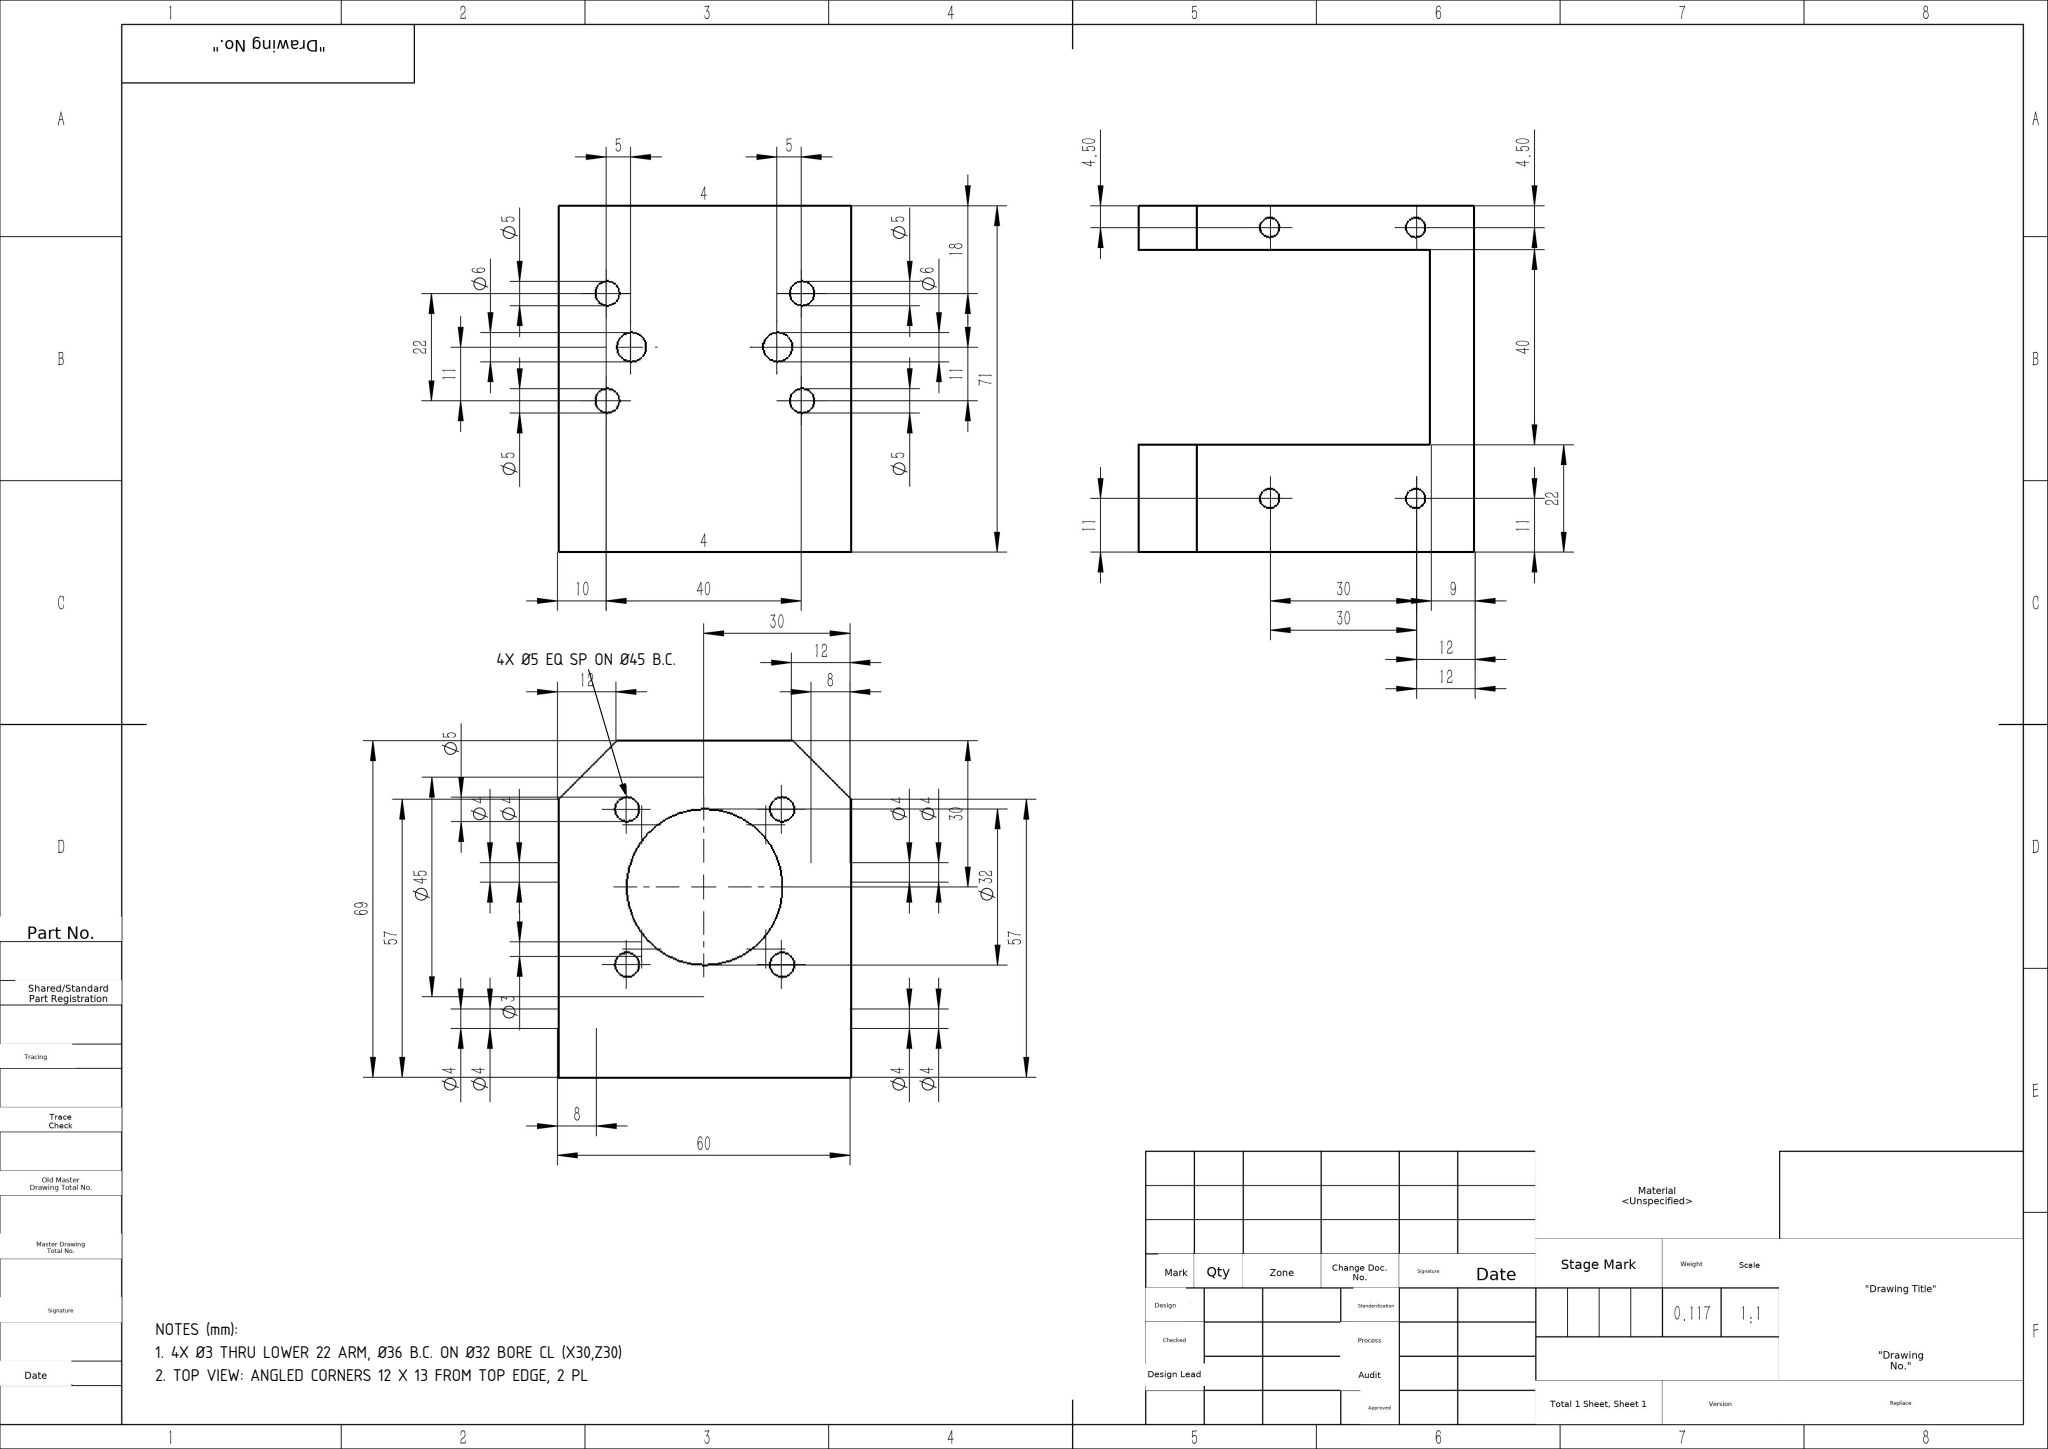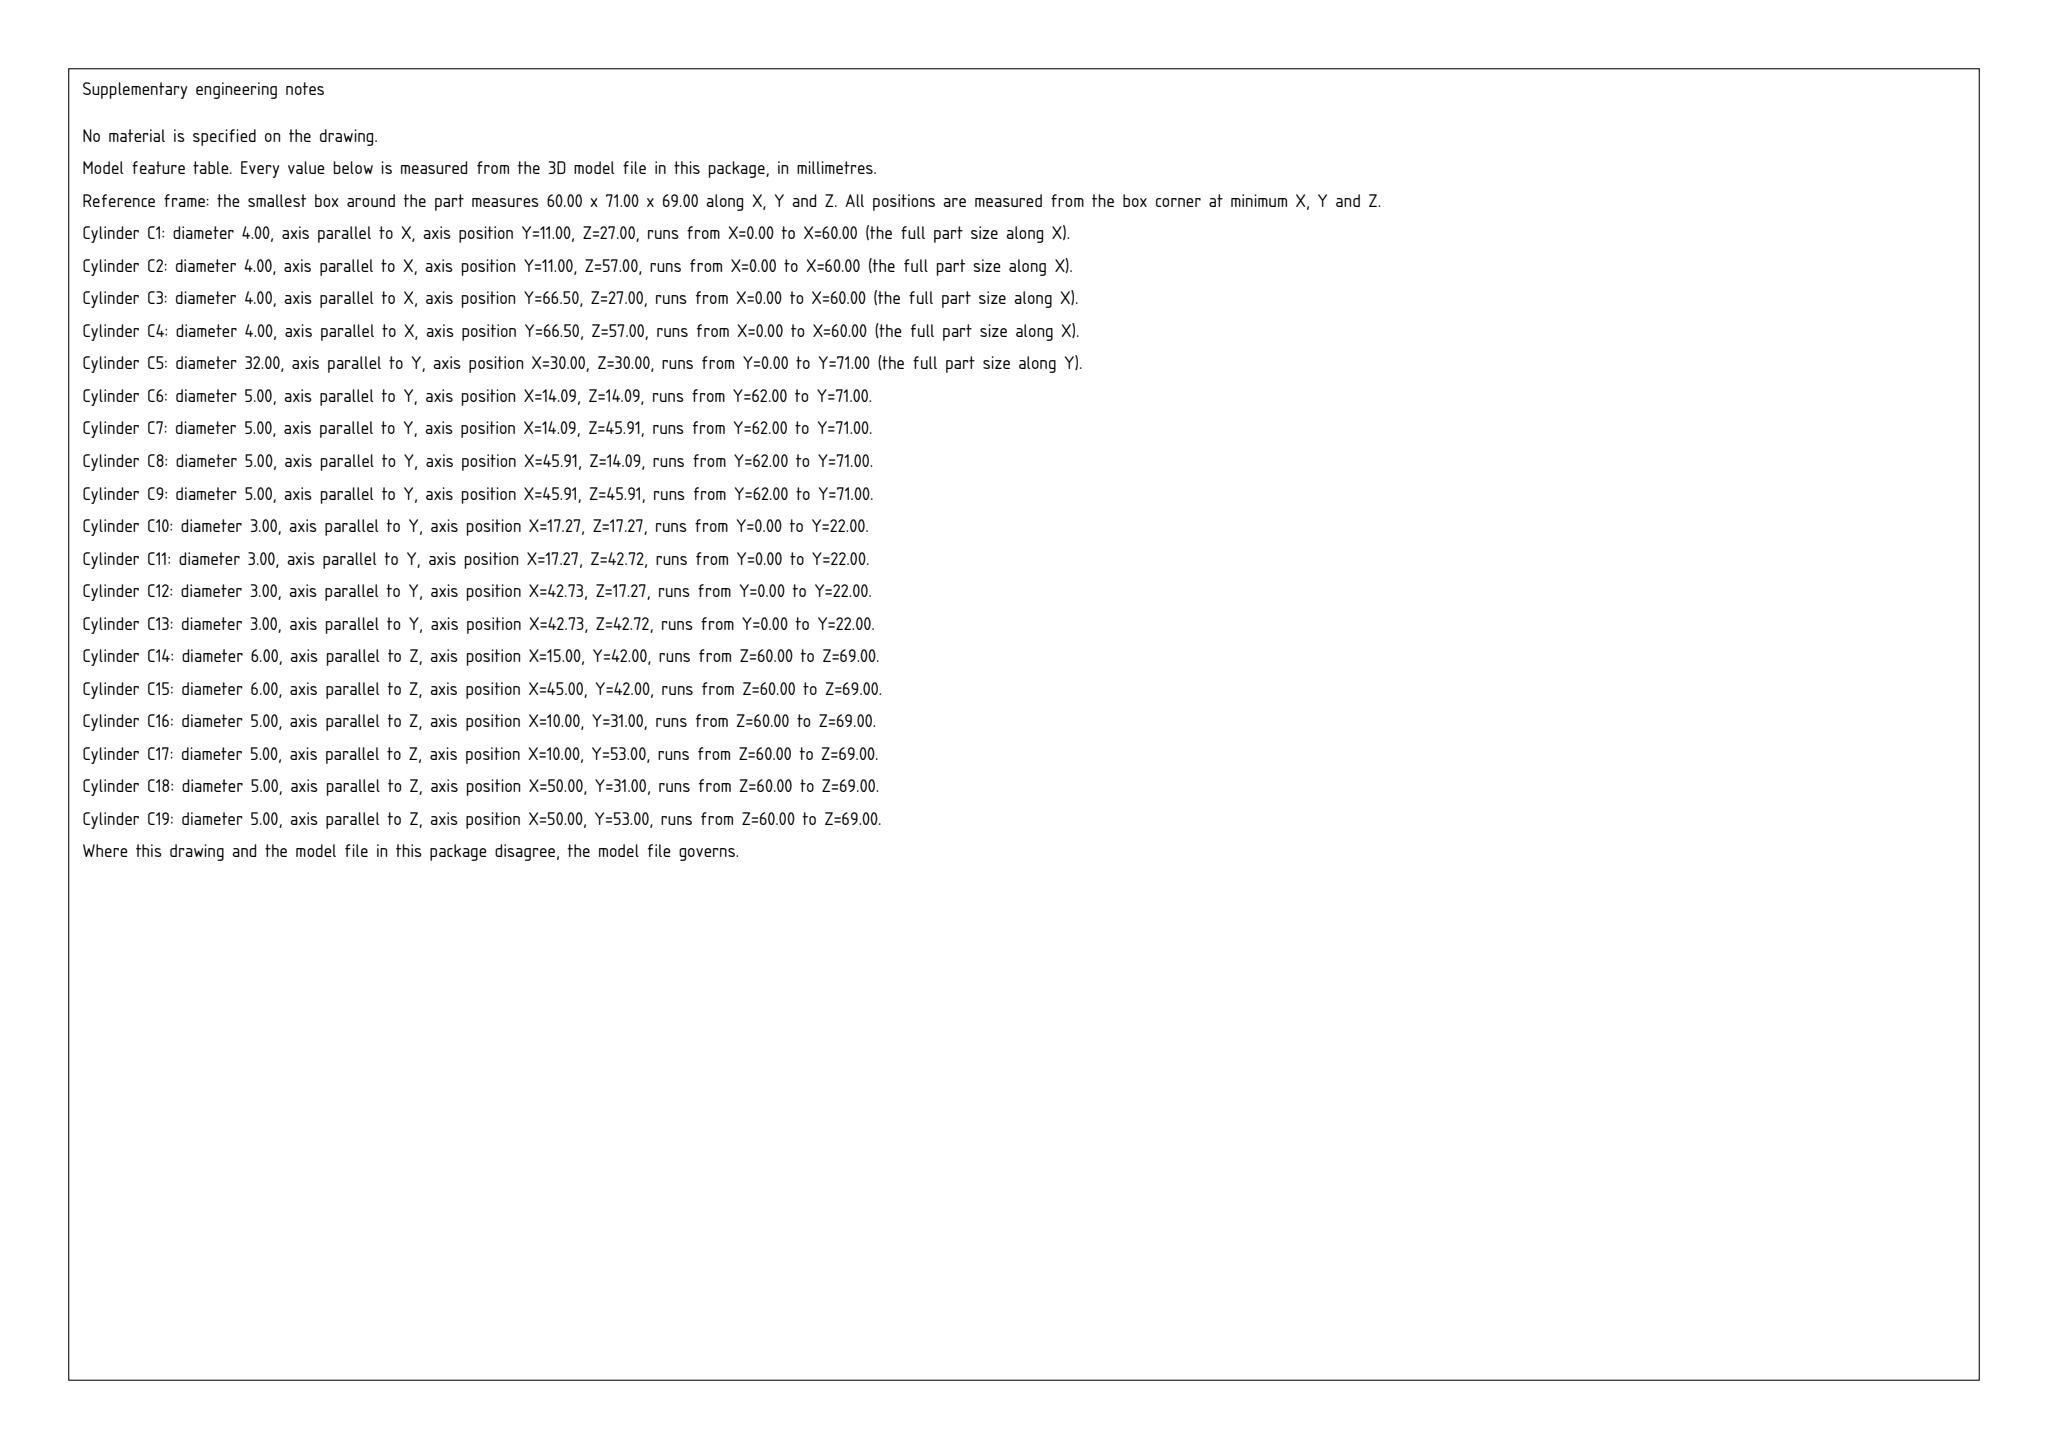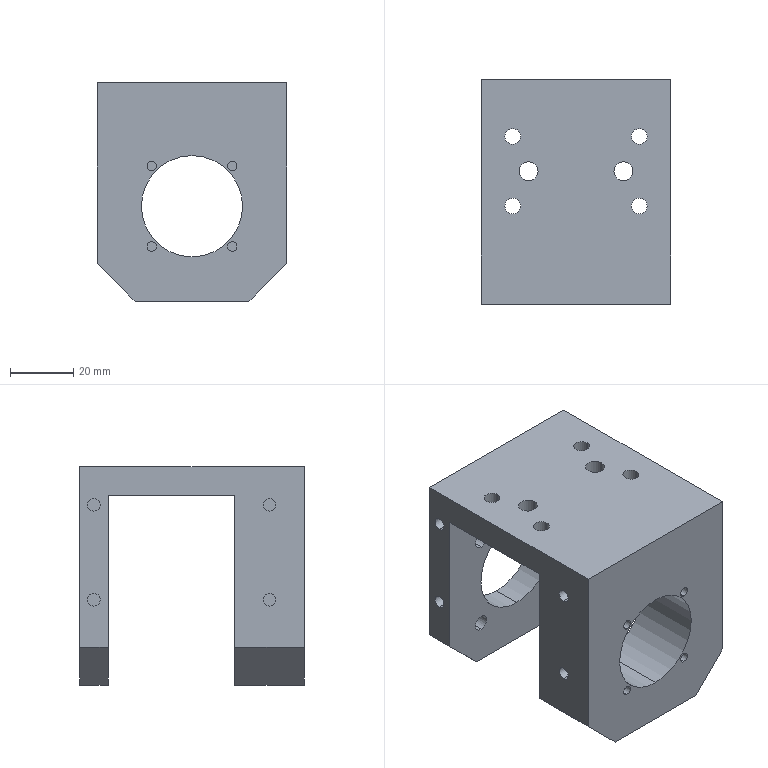Part | SolidWorks | mm | 1 solid | 70 faces | box 60 x 71 x 69 mm | volume 117195 mm3 | cylinder 48 | plane 22 | commonest cylinder face diameters 5 x16 4 x16 3 x8 6 x4 32 x4
Drawing notes:
4X Ø3 THRU LOWER 22 ARM, Ø36 B.C. ON Ø32 BORE CL (X30,Z30) | from the solid: Ø3 y-axis holes at (17.27/42.73, 17.27/42.73), L=22 (y 0-22 arm); radius from (30,30)=18 -> Ø36 B.C.
4X Ø5 ON Ø45 B.C. EQ SP 90°, CLOCKED 45°, B.C. CTR = Ø32 BORE CL | from the solid: Ø5 y-axis holes at (x,z)=(14.09,14.09),(14.09,45.91),(45.91,14.09),(45.91,45.91); CTR (30,30) = Ø32 y-bore axis; radius 22.5 at 45° increments, ↧9 (y 62-71)
TOP VIEW: ANGLED CORNERS 12 X 13 FROM TOP EDGE, 2 PL | from the solid: Upper arm 60 x 69 (x 0-60, z 0-69); straight side edges end 13 below z=69 face, cut runs 12 in X to the 36 wide top edge; no cone/fillet data
build123d program:
from build123d import *

# Parameters (mm, degrees)
BOSS_EXTRUDE1_DEPTH = 71
CUT_EXTRUDE1_REACH  = 101.668
SKETCH3_W           = 60
SKETCH3_H           = 40
CUT_EXTRUDE2_REACH  = 95.935
SKETCH4_R           = 16
SKETCH5_R           = 1.5
CUT_EXTRUDE3_DEPTH  = 62
SKETCH7_R           = 2.5
CUT_EXTRUDE4_DEPTH  = 49
SKETCH8_R           = 2
CUT_EXTRUDE5_DEPTH  = 8
CUT_EXTRUDE7_START  = -8
SKETCH9_R           = 2
CUT_EXTRUDE7_DEPTH  = 8
SKETCH10_R          = 2.5
SKETCH10_R_2        = 3
CUT_EXTRUDE8_DEPTH  = 9


with BuildPart() as part:
    # Sketch1 → Boss-Extrude1 (new body)
    with BuildSketch(Plane(origin=(0, 0, 0), x_dir=(1, 0, 0), z_dir=(0, 1, 0))):
        Polygon((-49.901, -33.046), (10.099, -33.046), (10.099, 23.954), (-1.901, 35.954), (-37.901, 35.954), (-49.901, 23.954), align=None)
    extrude(amount=BOSS_EXTRUDE1_DEPTH)

    # Cut-Extrude1: up to this face of the body (flat: up to its plane)
    cut_extrude1_end = Plane(part.part.faces().sort_by_distance((10.099, 35.5, 4.546))[0])
    # Sketch3 → Cut-Extrude1 (cut, up to the picked face)
    with BuildSketch(Plane.ZY.offset(49.901), mode=Mode.PRIVATE) as cut_extrude1_sk1:
        with Locations((-5.954, 42)):
            Rectangle(SKETCH3_W, SKETCH3_H)
    cut_extrude1_tool1 = split(extrude(cut_extrude1_sk1.sketch, amount=-CUT_EXTRUDE1_REACH, mode=Mode.PRIVATE), bisect_by=cut_extrude1_end, keep=Keep.BOTH, mode=Mode.PRIVATE)
    add(cut_extrude1_tool1.solids().sort_by(Axis((-49.901, 42, -5.954), (1, 0, 0)))[0], mode=Mode.SUBTRACT)

    # Cut-Extrude2: up to this face of the body (flat: up to its plane)
    cut_extrude2_end = Plane(part.part.faces().sort_by_distance((-19.901, 71, -0.3552))[0])
    # Sketch4 → Cut-Extrude2 (cut, up to the picked face)
    with BuildSketch(Plane.XZ, mode=Mode.PRIVATE) as cut_extrude2_sk1:
        with Locations(Location((-19.901, -5.954, 0), (0, 0, 270))):
            Circle(SKETCH4_R)
    cut_extrude2_tool1 = split(extrude(cut_extrude2_sk1.sketch, amount=-CUT_EXTRUDE2_REACH, mode=Mode.PRIVATE), bisect_by=cut_extrude2_end, keep=Keep.BOTH, mode=Mode.PRIVATE)
    add(cut_extrude2_tool1.solids().sort_by(Axis((-19.901, 0, -5.954), (0, 1, 0)))[0], mode=Mode.SUBTRACT)

    # Sketch5 → Cut-Extrude3 (cut)
    with BuildSketch(Plane.XZ):
        with Locations(Location((-32.628, 6.774, 0), (0, 0, 270))):
            Circle(SKETCH5_R)
        with Locations(Location((-7.173, 6.774, 0), (0, 0, 270))):
            Circle(SKETCH5_R)
        with Locations(Location((-7.173, -18.682, 0), (0, 0, 270))):
            Circle(SKETCH5_R)
        with Locations(Location((-32.628, -18.682, 0), (0, 0, 270))):
            Circle(SKETCH5_R)
    extrude(amount=-CUT_EXTRUDE3_DEPTH, mode=Mode.SUBTRACT)

    # Sketch7 → Cut-Extrude4 (cut)
    with BuildSketch(Plane(origin=(0, 71, 0), x_dir=(1, 0, 0), z_dir=(0, 1, 0))):
        with Locations(Location((-35.81, 21.864, 0), (0, 0, 270))):
            Circle(SKETCH7_R)
        with Locations(Location((-3.991, 21.864, 0), (0, 0, 270))):
            Circle(SKETCH7_R)
        with Locations(Location((-3.991, -9.956, 0), (0, 0, 270))):
            Circle(SKETCH7_R)
        with Locations(Location((-35.81, -9.956, 0), (0, 0, 270))):
            Circle(SKETCH7_R)
    extrude(amount=-CUT_EXTRUDE4_DEPTH, mode=Mode.SUBTRACT)

    # Sketch8 → Cut-Extrude5 (cut)
    with BuildSketch(Plane(origin=(10.099, 0, 0), x_dir=(0, 0, -1), z_dir=(1, 0, 0))):
        with Locations((-21.046, 66.5)):
            Circle(SKETCH8_R)
        with Locations((8.954, 66.5)):
            Circle(SKETCH8_R)
        with Locations((8.954, 11)):
            Circle(SKETCH8_R)
        with Locations((-21.046, 11)):
            Circle(SKETCH8_R)
    extrude(amount=-CUT_EXTRUDE5_DEPTH, mode=Mode.SUBTRACT)

    # Sketch9 → Cut-Extrude7 (cut)
    with BuildSketch(Plane.ZY.offset(49.901).offset(CUT_EXTRUDE7_START)):
        with Locations(Location((-8.954, 66.5, 0), (0, 0, 180))):
            Circle(SKETCH9_R)
        with Locations(Location((21.046, 66.5, 0), (0, 0, 180))):
            Circle(SKETCH9_R)
        with Locations(Location((-8.954, 11, 0), (0, 0, 180))):
            Circle(SKETCH9_R)
        with Locations(Location((21.046, 11, 0), (0, 0, 180))):
            Circle(SKETCH9_R)
    extrude(amount=CUT_EXTRUDE7_DEPTH, mode=Mode.SUBTRACT)

    # Sketch10 → Cut-Extrude8 (cut)
    with BuildSketch(Plane.XY.offset(33.046)):
        with Locations((-39.901, 53)):
            Circle(SKETCH10_R)
        with Locations((-39.901, 31)):
            Circle(SKETCH10_R)
        with Locations((0.09946, 31)):
            Circle(SKETCH10_R)
        with Locations((0.09946, 53)):
            Circle(SKETCH10_R)
        with Locations((-34.901, 42)):
            Circle(SKETCH10_R_2)
        with Locations((-4.901, 42)):
            Circle(SKETCH10_R_2)
    extrude(amount=-CUT_EXTRUDE8_DEPTH, mode=Mode.SUBTRACT)


solid = part.part